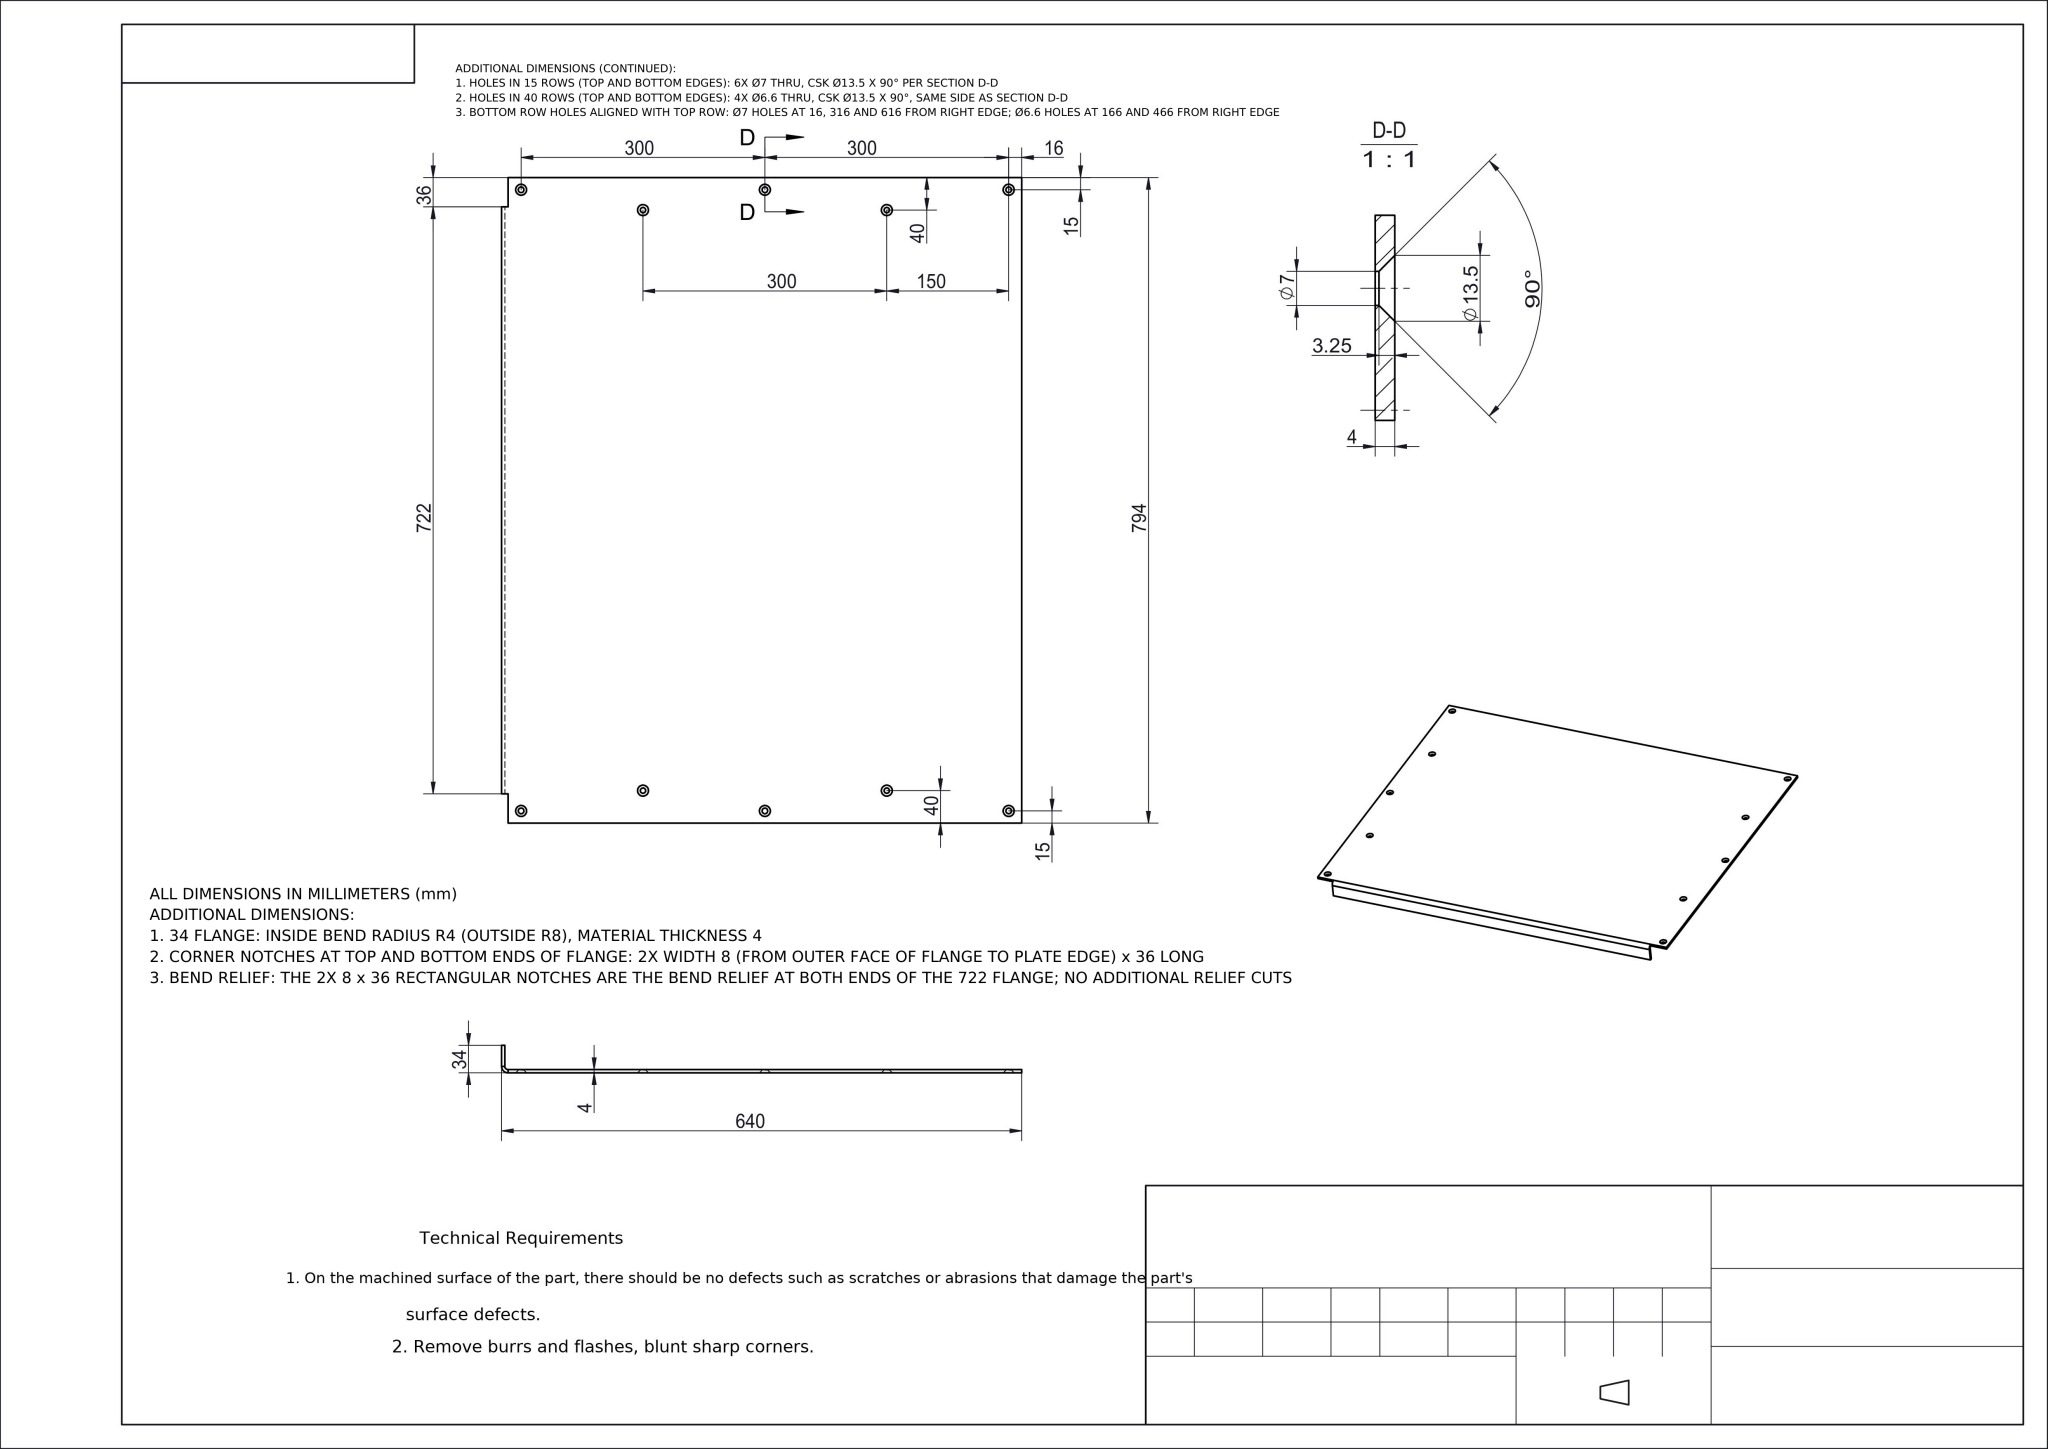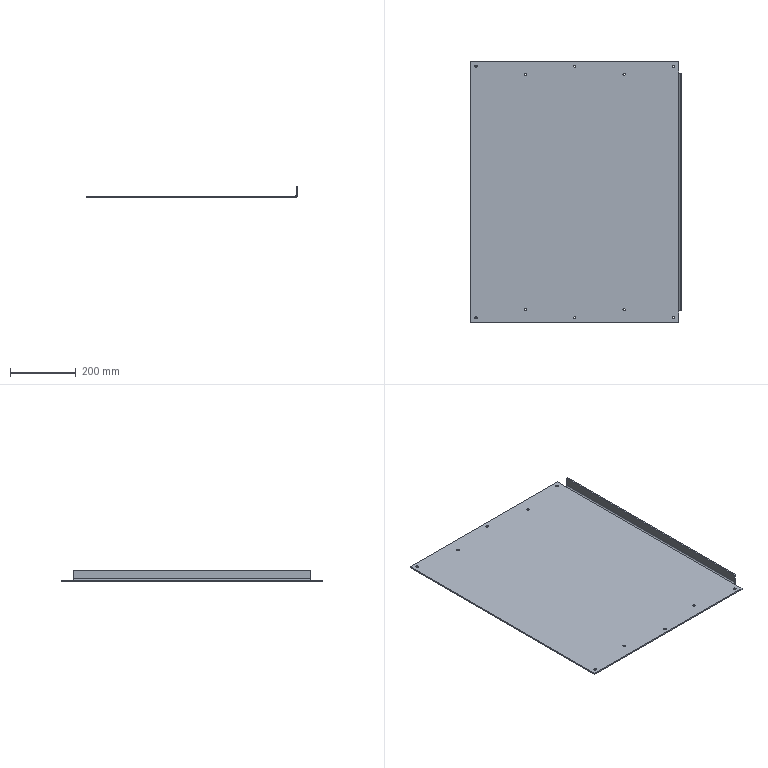Part | NX | mm | 1 solid | 56 faces | box 640 x 794 x 34 mm | volume 2106490 mm3 | cylinder 22 | cone 20 | plane 14 | commonest cylinder face diameters 7 x12 6.6 x8 16 x1 8 x1